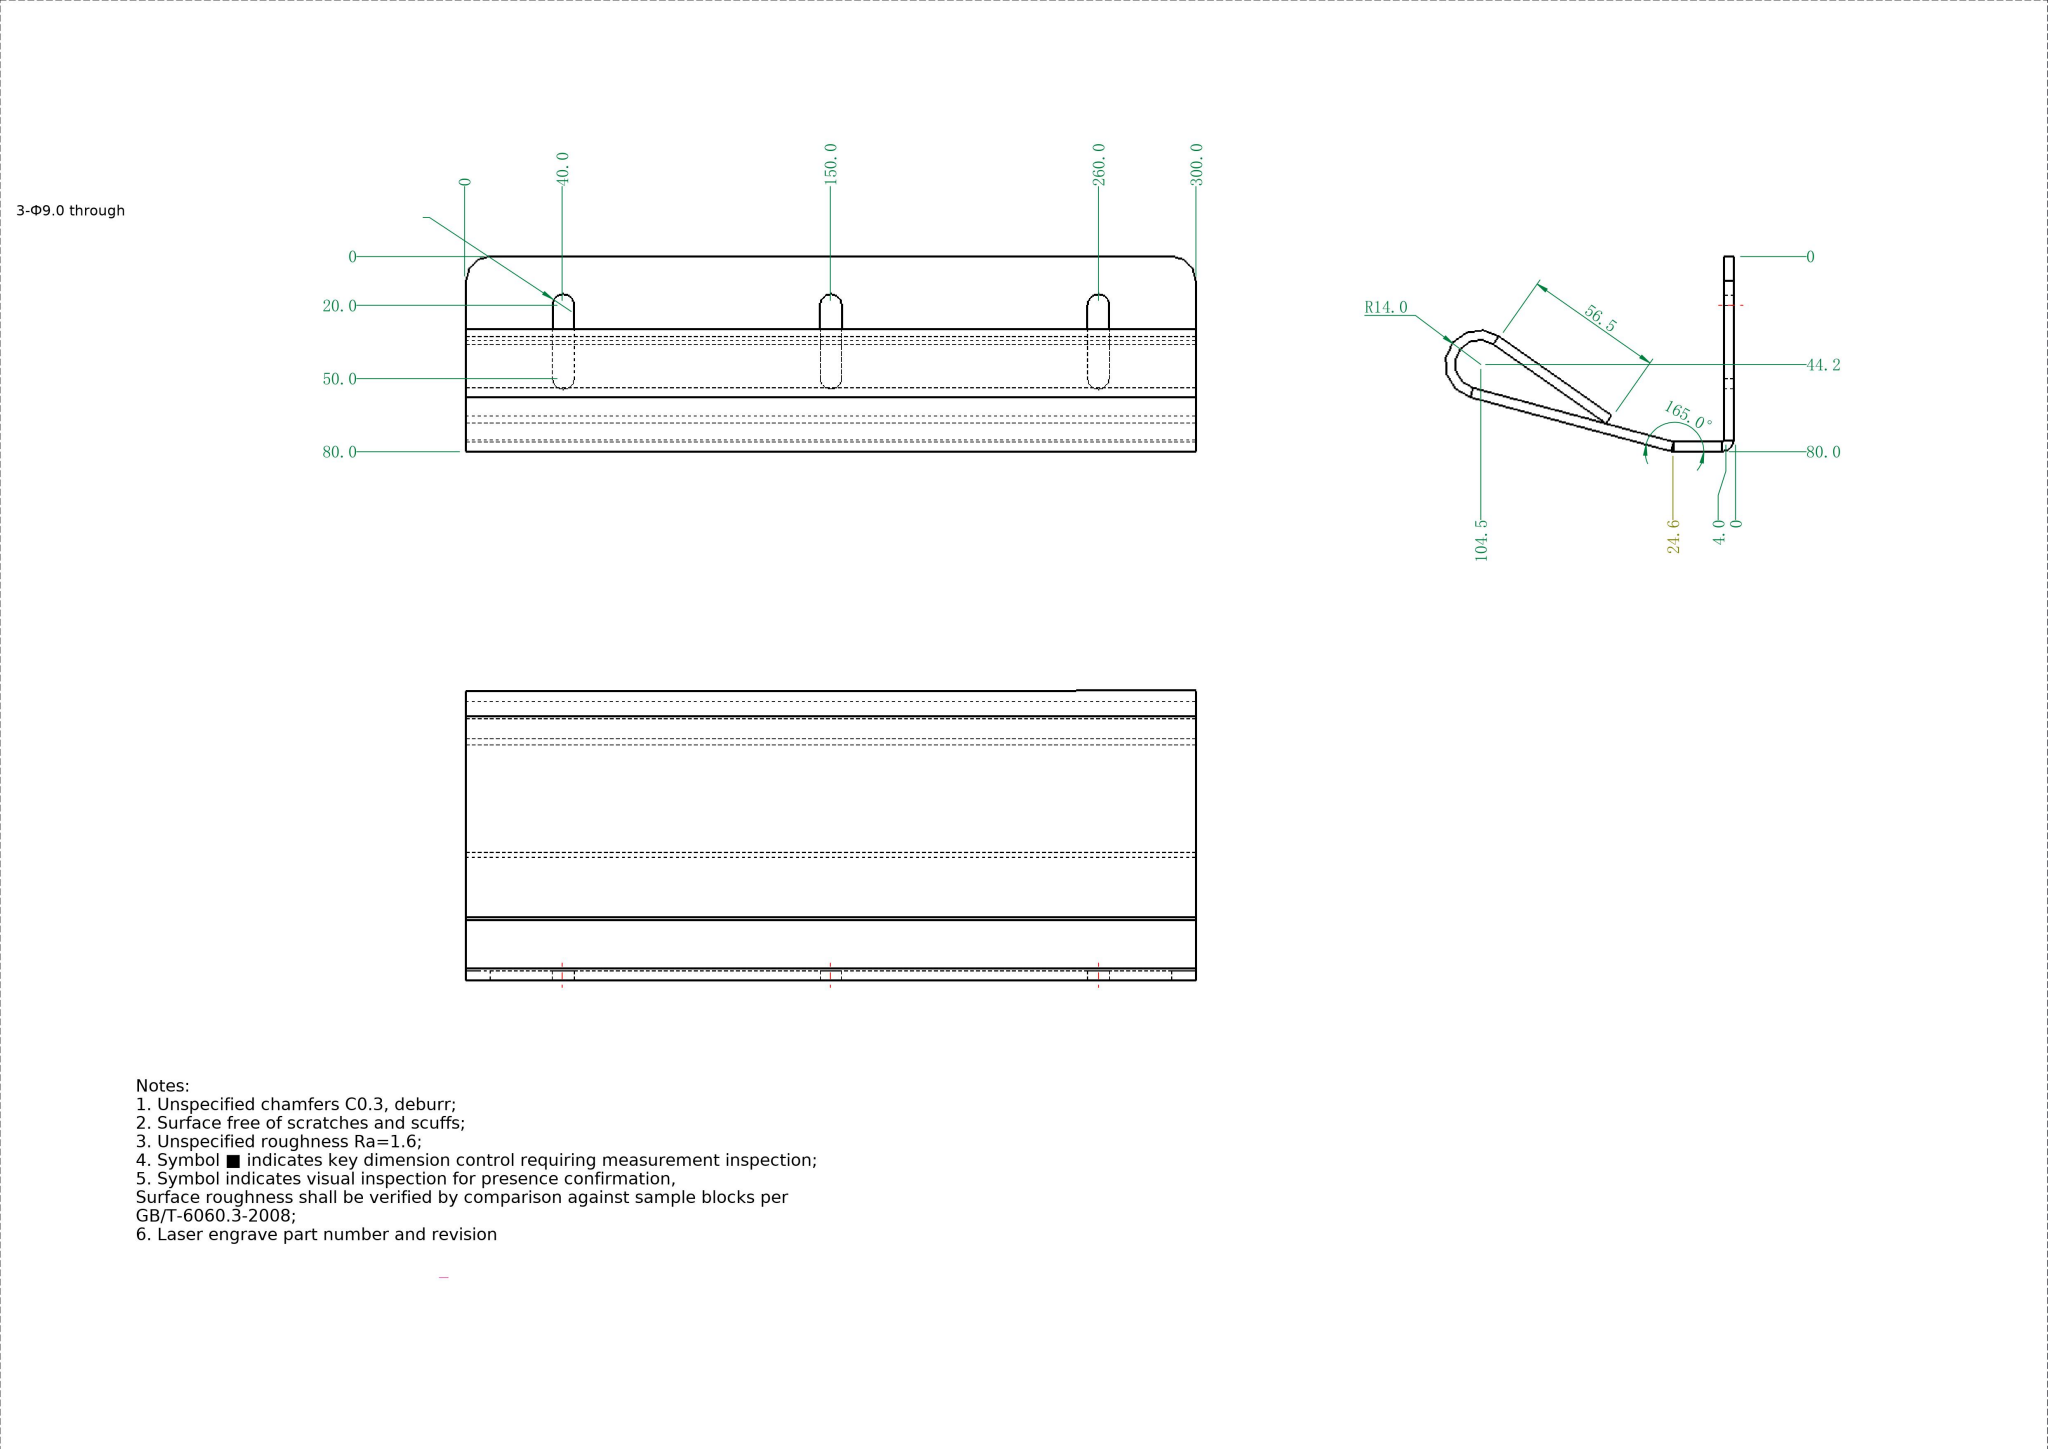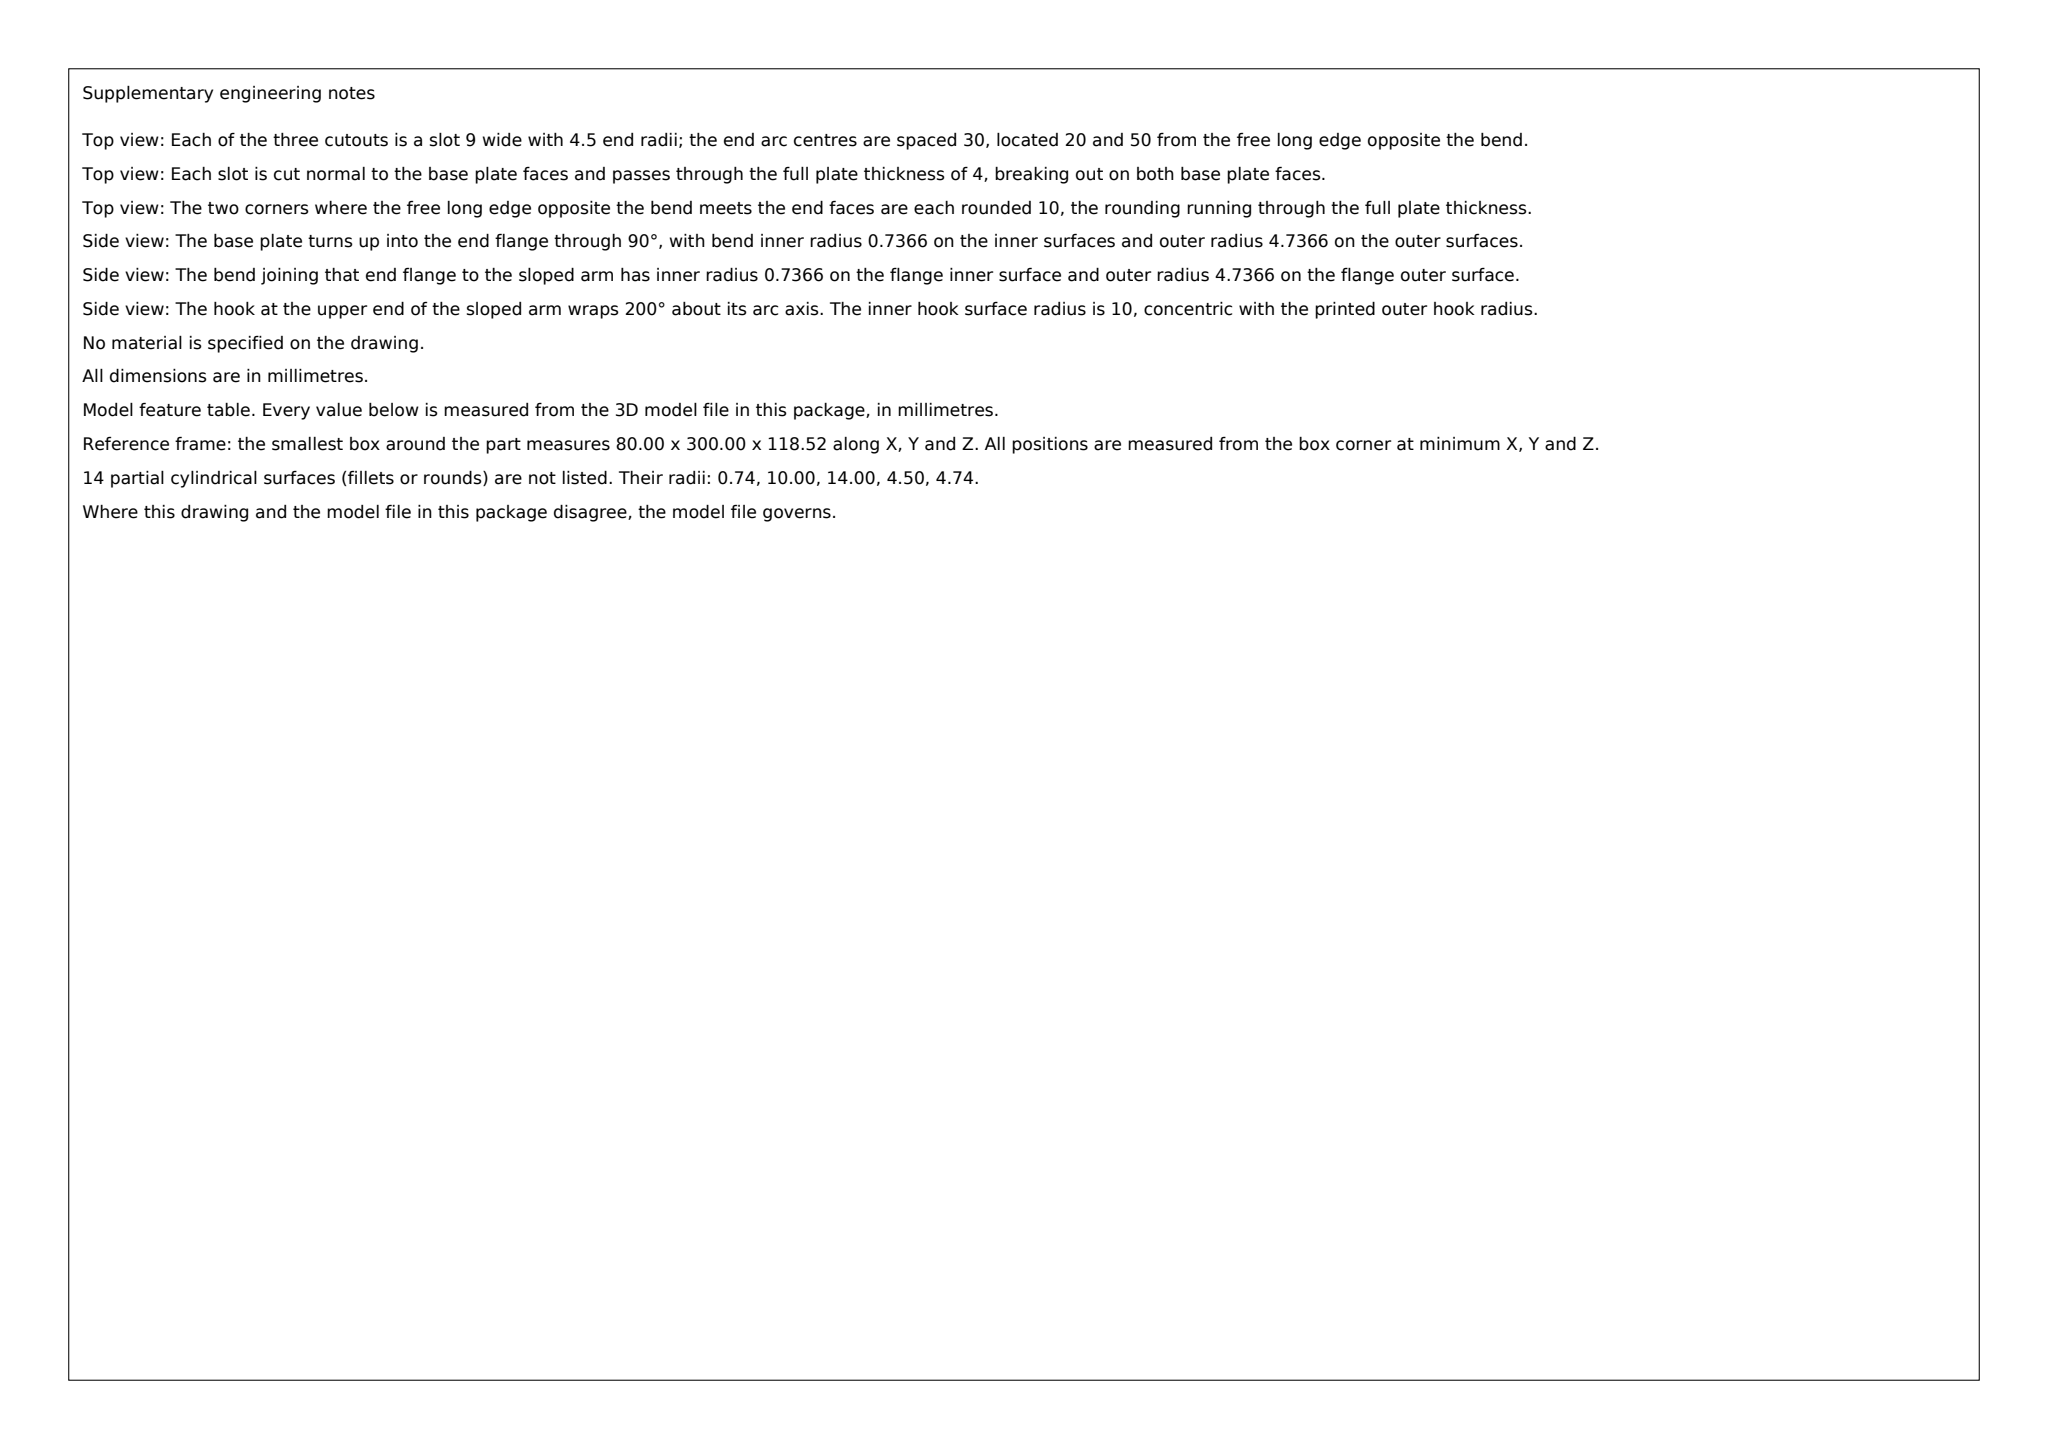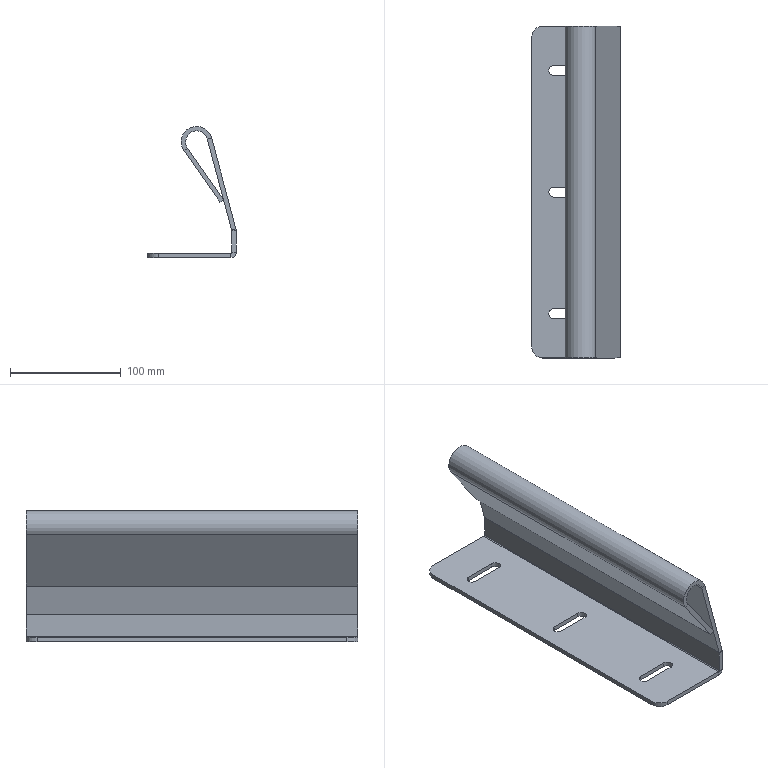Part | SolidWorks | mm | 1 solid | 44 faces | box 80 x 300 x 118.52 mm | volume 336346 mm3 | plane 30 | cylinder 14 | commonest cylinder face diameters 9 x6 20 x3 9.473 x2 1.473 x2 28 x1